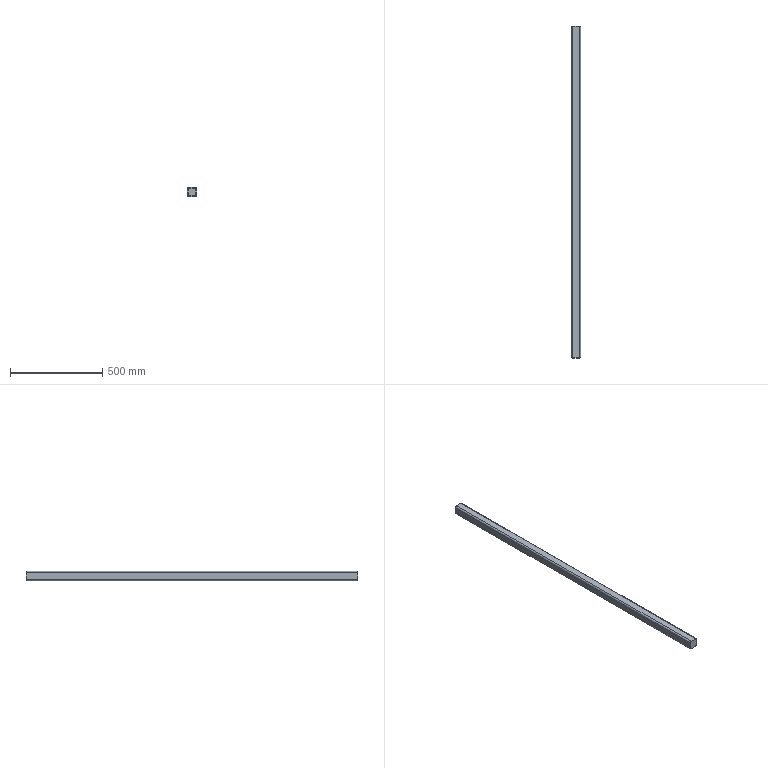Component | SolidWorks | AX00-100.1.1-1_AXFrame_A.1.1-1_AX50x50-3_square tube.1.1-3 | 1 solid | 20 faces | box 50 x 1800 x 50 mm | volume 1550940 mm3 | plane 12 | cylinder 8 | commonest cylinder face diameters 16 x4 6 x4 | material AISI 1035 Steel (SS)
build123d program:
from build123d import *

# Parameters (mm, degrees)
SKETCH1_W           = 50
SKETCH1_H           = 50
BOSS_EXTRUDE1_DEPTH = 900
FILLET3_R           = 8
SHELL1_T            = 5


with BuildPart() as part:
    # Sketch1 → Boss-Extrude1 (new, symmetric)
    with BuildSketch(Plane.XY):
        Rectangle(SKETCH1_W, SKETCH1_H)
    extrude(amount=BOSS_EXTRUDE1_DEPTH, both=True)

    # Fillet3
    fillet3_edges = [part.edges().sort_by_distance(p)[0] for p in [
        (25, -25, 0),
        (-25, -25, 0),
        (-25, 25, 0),
        (25, 25, 0),
    ]]
    fillet(fillet3_edges, radius=FILLET3_R)

    # Shell1 (no face opened: a closed hollow body)
    add(offset(amount=-SHELL1_T, mode=Mode.PRIVATE), mode=Mode.SUBTRACT)


solid = part.part

# Placed as in the assembly
solid = solid.moved(Location((1143.631, 563.364, 187.5), (90, 0, 0)))